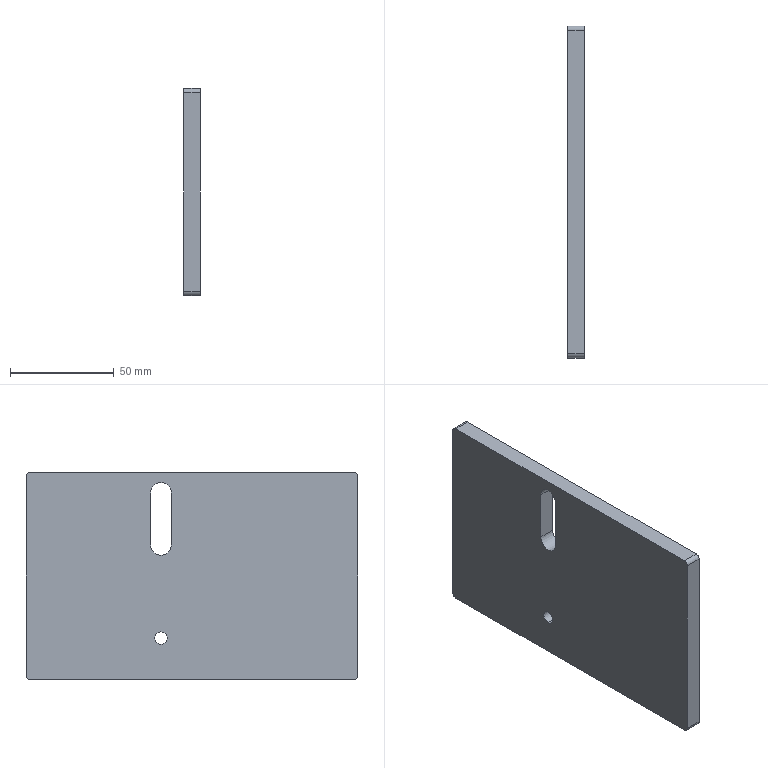Component | SolidWorks | CHEN123-AA-11-1 | 1 solid | 17 faces | box 8 x 160 x 100 mm | volume 125118 mm3 | cylinder 9 | plane 8 | commonest cylinder face diameters 4 x4 10 x3 6 x2
build123d program:
from build123d import *

# Parameters (mm, degrees)
SKETCH1_W           = 100
SKETCH1_H           = 160
BOSS_EXTRUDE1_DEPTH = 8
FILLET1_R           = 2
CUT_EXTRUDE1_DEPTH  = 95.678
SKETCH3_R           = 3
CUT_EXTRUDE2_DEPTH  = 95.678


with BuildPart() as part:
    # Sketch1 → Boss-Extrude1 (new body)
    with BuildSketch(Plane.XY):
        Rectangle(SKETCH1_W, SKETCH1_H)
    extrude(amount=BOSS_EXTRUDE1_DEPTH)

    # Fillet1
    fillet1_edges = [part.edges().sort_by_distance(p)[0] for p in [
        (50, -80, 4),
        (-50, -80, 4),
        (-50, 80, 4),
        (50, 80, 4),
    ]]
    fillet(fillet1_edges, radius=FILLET1_R)

    # Sketch2 → Cut-Extrude1 (cut, through all)
    with BuildSketch(Plane.XY.offset(8)):
        with BuildLine():
            Line((15, 10), (40, 10))
            ThreePointArc((40, 10), (45, 15), (40, 20))
            Line((40, 20), (15, 20))
            ThreePointArc((15, 20), (10, 15), (15, 10))
        make_face()
    extrude(amount=-CUT_EXTRUDE1_DEPTH, mode=Mode.SUBTRACT)

    # Sketch3 → Cut-Extrude2 (cut, through all)
    with BuildSketch(Plane(origin=(0, 0, 0), x_dir=(-1, 0, 0), z_dir=(0, 0, -1))):
        with Locations((30, 15)):
            Circle(SKETCH3_R)
    extrude(amount=-CUT_EXTRUDE2_DEPTH, mode=Mode.SUBTRACT)


solid = part.part

# Placed as in the assembly
solid = solid.moved(Location((28, -60.999, -200), (0, -90, 0)))
STEP:
#1=COLOUR_RGB('',0.7922,0.8196,0.9333);
#2=FILL_AREA_STYLE_COLOUR('',#1);
#3=FILL_AREA_STYLE('',(#2));
#4=SURFACE_STYLE_FILL_AREA(#3);
#5=SURFACE_SIDE_STYLE('',(#4));
#6=SURFACE_STYLE_USAGE(.BOTH.,#5);
#7=PRESENTATION_STYLE_ASSIGNMENT((#6));
#8=CARTESIAN_POINT('',(0.7874,-1.811,-8.937));
#9=VERTEX_POINT('',#8);
#10=CARTESIAN_POINT('',(0.7874,-1.811,-9.173));
#11=VERTEX_POINT('',#10);
#12=CARTESIAN_POINT('',(0.7874,-1.811,-9.055));
#13=DIRECTION('',(1.,0.,0.));
#14=DIRECTION('',(0.,0.,-1.));
#15=AXIS2_PLACEMENT_3D('',#12,#13,#14);
#16=CIRCLE('',#15,0.1181);
#17=EDGE_CURVE('',#9,#11,#16,.T.);
#18=ORIENTED_EDGE('',*,*,#17,.F.);
#19=CARTESIAN_POINT('',(1.102,-1.811,-8.937));
#20=VERTEX_POINT('',#19);
#21=CARTESIAN_POINT('',(0.7874,-1.811,-8.937));
#22=DIRECTION('',(1.,0.,0.));
#23=VECTOR('',#22,39.37);
#24=LINE('',#21,#23);
#25=EDGE_CURVE('',#9,#20,#24,.T.);
#26=ORIENTED_EDGE('',*,*,#25,.T.);
#27=CARTESIAN_POINT('',(1.102,-1.811,-9.173));
#28=VERTEX_POINT('',#27);
#29=CARTESIAN_POINT('',(1.102,-1.811,-9.055));
#30=DIRECTION('',(1.,0.,0.));
#31=DIRECTION('',(0.,0.,-1.));
#32=AXIS2_PLACEMENT_3D('',#29,#30,#31);
#33=CIRCLE('',#32,0.1181);
#34=EDGE_CURVE('',#20,#28,#33,.T.);
#35=ORIENTED_EDGE('',*,*,#34,.T.);
#36=CARTESIAN_POINT('',(0.7874,-1.811,-9.173));
#37=DIRECTION('',(1.,0.,0.));
#38=VECTOR('',#37,39.37);
#39=LINE('',#36,#38);
#40=EDGE_CURVE('',#11,#28,#39,.T.);
#41=ORIENTED_EDGE('',*,*,#40,.F.);
#42=EDGE_LOOP('',(#18,#26,#35,#41));
#43=FACE_OUTER_BOUND('',#42,.T.);
#44=CARTESIAN_POINT('',(0.7874,-1.811,-9.055));
#45=DIRECTION('',(1.,0.,0.));
#46=DIRECTION('',(0.,0.,-1.));
#47=AXIS2_PLACEMENT_3D('',#44,#45,#46);
#48=CYLINDRICAL_SURFACE('',#47,0.1181);
#49=ADVANCED_FACE('',(#43),#48,.F.);
#50=CARTESIAN_POINT('',(1.102,-1.811,-6.102));
#51=VERTEX_POINT('',#50);
#52=CARTESIAN_POINT('',(1.102,-1.614,-6.299));
#53=VERTEX_POINT('',#52);
#54=CARTESIAN_POINT('',(1.102,-1.811,-6.299));
#55=DIRECTION('',(-1.,0.,0.));
#56=DIRECTION('',(0.,0.,1.));
#57=AXIS2_PLACEMENT_3D('',#54,#55,#56);
#58=CIRCLE('',#57,0.1969);
#59=EDGE_CURVE('',#51,#53,#58,.T.);
#60=ORIENTED_EDGE('',*,*,#59,.F.);
#61=CARTESIAN_POINT('',(0.7874,-1.811,-6.102));
#62=VERTEX_POINT('',#61);
#63=CARTESIAN_POINT('',(1.102,-1.811,-6.102));
#64=DIRECTION('',(-1.,0.,0.));
#65=VECTOR('',#64,39.37);
#66=LINE('',#63,#65);
#67=EDGE_CURVE('',#51,#62,#66,.T.);
#68=ORIENTED_EDGE('',*,*,#67,.T.);
#69=CARTESIAN_POINT('',(0.7874,-1.614,-6.299));
#70=VERTEX_POINT('',#69);
#71=CARTESIAN_POINT('',(0.7874,-1.811,-6.299));
#72=DIRECTION('',(-1.,0.,0.));
#73=DIRECTION('',(0.,0.,1.));
#74=AXIS2_PLACEMENT_3D('',#71,#72,#73);
#75=CIRCLE('',#74,0.1969);
#76=EDGE_CURVE('',#62,#70,#75,.T.);
#77=ORIENTED_EDGE('',*,*,#76,.T.);
#78=CARTESIAN_POINT('',(1.102,-1.614,-6.299));
#79=DIRECTION('',(-1.,0.,0.));
#80=VECTOR('',#79,39.37);
#81=LINE('',#78,#80);
#82=EDGE_CURVE('',#53,#70,#81,.T.);
#83=ORIENTED_EDGE('',*,*,#82,.F.);
#84=EDGE_LOOP('',(#60,#68,#77,#83));
#85=FACE_OUTER_BOUND('',#84,.T.);
#86=CARTESIAN_POINT('',(1.102,-1.811,-6.299));
#87=DIRECTION('',(-1.,0.,0.));
#88=DIRECTION('',(0.,0.,1.));
#89=AXIS2_PLACEMENT_3D('',#86,#87,#88);
#90=CYLINDRICAL_SURFACE('',#89,0.1969);
#91=ADVANCED_FACE('',(#85),#90,.F.);
#92=CARTESIAN_POINT('',(0.7874,-5.472,-5.906));
#93=VERTEX_POINT('',#92);
#94=CARTESIAN_POINT('',(0.7874,0.6693,-5.906));
#95=VERTEX_POINT('',#94);
#96=CARTESIAN_POINT('',(0.7874,-5.551,-5.906));
#97=DIRECTION('',(0.,1.,0.));
#98=VECTOR('',#97,39.37);
#99=LINE('',#96,#98);
#100=EDGE_CURVE('',#93,#95,#99,.T.);
#101=ORIENTED_EDGE('',*,*,#100,.F.);
#102=CARTESIAN_POINT('',(1.102,-5.472,-5.906));
#103=VERTEX_POINT('',#102);
#104=CARTESIAN_POINT('',(0.7874,-5.472,-5.906));
#105=DIRECTION('',(1.,0.,0.));
#106=VECTOR('',#105,39.37);
#107=LINE('',#104,#106);
#108=EDGE_CURVE('',#93,#103,#107,.T.);
#109=ORIENTED_EDGE('',*,*,#108,.T.);
#110=CARTESIAN_POINT('',(1.102,0.6693,-5.906));
#111=VERTEX_POINT('',#110);
#112=CARTESIAN_POINT('',(1.102,-5.551,-5.906));
#113=DIRECTION('',(0.,1.,0.));
#114=VECTOR('',#113,39.37);
#115=LINE('',#112,#114);
#116=EDGE_CURVE('',#103,#111,#115,.T.);
#117=ORIENTED_EDGE('',*,*,#116,.T.);
#118=CARTESIAN_POINT('',(0.7874,0.6693,-5.906));
#119=DIRECTION('',(-1.,0.,0.));
#120=VECTOR('',#119,39.37);
#121=LINE('',#118,#120);
#122=EDGE_CURVE('',#111,#95,#121,.T.);
#123=ORIENTED_EDGE('',*,*,#122,.T.);
#124=EDGE_LOOP('',(#101,#109,#117,#123));
#125=FACE_OUTER_BOUND('',#124,.T.);
#126=CARTESIAN_POINT('',(0.7874,-5.551,-5.906));
#127=DIRECTION('',(0.,0.,-1.));
#128=DIRECTION('',(-1.,0.,0.));
#129=AXIS2_PLACEMENT_3D('',#126,#127,#128);
#130=PLANE('',#129);
#131=ADVANCED_FACE('',(#125),#130,.F.);
#132=CARTESIAN_POINT('',(0.7874,0.7481,-5.984));
#133=VERTEX_POINT('',#132);
#134=CARTESIAN_POINT('',(0.7874,0.7481,-9.764));
#135=VERTEX_POINT('',#134);
#136=CARTESIAN_POINT('',(0.7874,0.7481,-9.843));
#137=DIRECTION('',(0.,0.,-1.));
#138=VECTOR('',#137,39.37);
#139=LINE('',#136,#138);
#140=EDGE_CURVE('',#133,#135,#139,.T.);
#141=ORIENTED_EDGE('',*,*,#140,.F.);
#142=CARTESIAN_POINT('',(1.102,0.7481,-5.984));
#143=VERTEX_POINT('',#142);
#144=CARTESIAN_POINT('',(0.7874,0.7481,-5.984));
#145=DIRECTION('',(1.,0.,0.));
#146=VECTOR('',#145,39.37);
#147=LINE('',#144,#146);
#148=EDGE_CURVE('',#133,#143,#147,.T.);
#149=ORIENTED_EDGE('',*,*,#148,.T.);
#150=CARTESIAN_POINT('',(1.102,0.7481,-9.764));
#151=VERTEX_POINT('',#150);
#152=CARTESIAN_POINT('',(1.102,0.7481,-9.843));
#153=DIRECTION('',(0.,0.,-1.));
#154=VECTOR('',#153,39.37);
#155=LINE('',#152,#154);
#156=EDGE_CURVE('',#143,#151,#155,.T.);
#157=ORIENTED_EDGE('',*,*,#156,.T.);
#158=CARTESIAN_POINT('',(0.7874,0.7481,-9.764));
#159=DIRECTION('',(-1.,0.,0.));
#160=VECTOR('',#159,39.37);
#161=LINE('',#158,#160);
#162=EDGE_CURVE('',#151,#135,#161,.T.);
#163=ORIENTED_EDGE('',*,*,#162,.T.);
#164=EDGE_LOOP('',(#141,#149,#157,#163));
#165=FACE_OUTER_BOUND('',#164,.T.);
#166=CARTESIAN_POINT('',(0.7874,0.7481,-9.843));
#167=DIRECTION('',(0.,-1.,0.));
#168=DIRECTION('',(1.,0.,0.));
#169=AXIS2_PLACEMENT_3D('',#166,#167,#168);
#170=PLANE('',#169);
#171=ADVANCED_FACE('',(#165),#170,.F.);
#172=CARTESIAN_POINT('',(1.102,0.6693,-9.843));
#173=VERTEX_POINT('',#172);
#174=CARTESIAN_POINT('',(1.102,-5.472,-9.843));
#175=VERTEX_POINT('',#174);
#176=CARTESIAN_POINT('',(1.102,-5.551,-9.843));
#177=DIRECTION('',(0.,-1.,0.));
#178=VECTOR('',#177,39.37);
#179=LINE('',#176,#178);
#180=EDGE_CURVE('',#173,#175,#179,.T.);
#181=ORIENTED_EDGE('',*,*,#180,.T.);
#182=CARTESIAN_POINT('',(0.7874,-5.472,-9.843));
#183=VERTEX_POINT('',#182);
#184=CARTESIAN_POINT('',(0.7874,-5.472,-9.843));
#185=DIRECTION('',(-1.,0.,0.));
#186=VECTOR('',#185,39.37);
#187=LINE('',#184,#186);
#188=EDGE_CURVE('',#175,#183,#187,.T.);
#189=ORIENTED_EDGE('',*,*,#188,.T.);
#190=CARTESIAN_POINT('',(0.7874,0.6693,-9.843));
#191=VERTEX_POINT('',#190);
#192=CARTESIAN_POINT('',(0.7874,-5.551,-9.843));
#193=DIRECTION('',(0.,-1.,0.));
#194=VECTOR('',#193,39.37);
#195=LINE('',#192,#194);
#196=EDGE_CURVE('',#191,#183,#195,.T.);
#197=ORIENTED_EDGE('',*,*,#196,.F.);
#198=CARTESIAN_POINT('',(0.7874,0.6693,-9.843));
#199=DIRECTION('',(1.,0.,0.));
#200=VECTOR('',#199,39.37);
#201=LINE('',#198,#200);
#202=EDGE_CURVE('',#191,#173,#201,.T.);
#203=ORIENTED_EDGE('',*,*,#202,.T.);
#204=EDGE_LOOP('',(#181,#189,#197,#203));
#205=FACE_OUTER_BOUND('',#204,.T.);
#206=CARTESIAN_POINT('',(0.7874,-5.551,-9.843));
#207=DIRECTION('',(0.,0.,1.));
#208=DIRECTION('',(1.,0.,0.));
#209=AXIS2_PLACEMENT_3D('',#206,#207,#208);
#210=PLANE('',#209);
#211=ADVANCED_FACE('',(#205),#210,.F.);
#212=CARTESIAN_POINT('',(1.102,-5.551,-9.764));
#213=VERTEX_POINT('',#212);
#214=CARTESIAN_POINT('',(1.102,-5.551,-5.984));
#215=VERTEX_POINT('',#214);
#216=CARTESIAN_POINT('',(1.102,-5.551,-9.843));
#217=DIRECTION('',(0.,0.,1.));
#218=VECTOR('',#217,39.37);
#219=LINE('',#216,#218);
#220=EDGE_CURVE('',#213,#215,#219,.T.);
#221=ORIENTED_EDGE('',*,*,#220,.T.);
#222=CARTESIAN_POINT('',(0.7874,-5.551,-5.984));
#223=VERTEX_POINT('',#222);
#224=CARTESIAN_POINT('',(0.7874,-5.551,-5.984));
#225=DIRECTION('',(-1.,0.,0.));
#226=VECTOR('',#225,39.37);
#227=LINE('',#224,#226);
#228=EDGE_CURVE('',#215,#223,#227,.T.);
#229=ORIENTED_EDGE('',*,*,#228,.T.);
#230=CARTESIAN_POINT('',(0.7874,-5.551,-9.764));
#231=VERTEX_POINT('',#230);
#232=CARTESIAN_POINT('',(0.7874,-5.551,-9.843));
#233=DIRECTION('',(0.,0.,1.));
#234=VECTOR('',#233,39.37);
#235=LINE('',#232,#234);
#236=EDGE_CURVE('',#231,#223,#235,.T.);
#237=ORIENTED_EDGE('',*,*,#236,.F.);
#238=CARTESIAN_POINT('',(0.7874,-5.551,-9.764));
#239=DIRECTION('',(1.,0.,0.));
#240=VECTOR('',#239,39.37);
#241=LINE('',#238,#240);
#242=EDGE_CURVE('',#231,#213,#241,.T.);
#243=ORIENTED_EDGE('',*,*,#242,.T.);
#244=EDGE_LOOP('',(#221,#229,#237,#243));
#245=FACE_OUTER_BOUND('',#244,.T.);
#246=CARTESIAN_POINT('',(0.7874,-5.551,-9.843));
#247=DIRECTION('',(0.,1.,0.));
#248=DIRECTION('',(-1.,0.,0.));
#249=AXIS2_PLACEMENT_3D('',#246,#247,#248);
#250=PLANE('',#249);
#251=ADVANCED_FACE('',(#245),#250,.F.);
#252=CARTESIAN_POINT('',(0.7874,-1.811,-9.055));
#253=DIRECTION('',(1.,0.,0.));
#254=DIRECTION('',(0.,0.,-1.));
#255=AXIS2_PLACEMENT_3D('',#252,#253,#254);
#256=CIRCLE('',#255,0.1181);
#257=EDGE_CURVE('',#11,#9,#256,.T.);
#258=ORIENTED_EDGE('',*,*,#257,.T.);
#259=ORIENTED_EDGE('',*,*,#17,.T.);
#260=EDGE_LOOP('',(#258,#259));
#261=FACE_BOUND('',#260,.T.);
#262=CARTESIAN_POINT('',(0.7874,-1.614,-7.283));
#263=VERTEX_POINT('',#262);
#264=CARTESIAN_POINT('',(0.7874,-1.614,-6.299));
#265=DIRECTION('',(0.,0.,-1.));
#266=VECTOR('',#265,39.37);
#267=LINE('',#264,#266);
#268=EDGE_CURVE('',#70,#263,#267,.T.);
#269=ORIENTED_EDGE('',*,*,#268,.F.);
#270=ORIENTED_EDGE('',*,*,#76,.F.);
#271=CARTESIAN_POINT('',(0.7874,-2.008,-6.299));
#272=VERTEX_POINT('',#271);
#273=CARTESIAN_POINT('',(0.7874,-1.811,-6.299));
#274=DIRECTION('',(-1.,0.,0.));
#275=DIRECTION('',(0.,0.,1.));
#276=AXIS2_PLACEMENT_3D('',#273,#274,#275);
#277=CIRCLE('',#276,0.1969);
#278=EDGE_CURVE('',#272,#62,#277,.T.);
#279=ORIENTED_EDGE('',*,*,#278,.F.);
#280=CARTESIAN_POINT('',(0.7874,-2.008,-7.283));
#281=VERTEX_POINT('',#280);
#282=CARTESIAN_POINT('',(0.7874,-2.008,-7.283));
#283=DIRECTION('',(0.,0.,1.));
#284=VECTOR('',#283,39.37);
#285=LINE('',#282,#284);
#286=EDGE_CURVE('',#281,#272,#285,.T.);
#287=ORIENTED_EDGE('',*,*,#286,.F.);
#288=CARTESIAN_POINT('',(0.7874,-1.811,-7.283));
#289=DIRECTION('',(-1.,0.,0.));
#290=DIRECTION('',(0.,0.,1.));
#291=AXIS2_PLACEMENT_3D('',#288,#289,#290);
#292=CIRCLE('',#291,0.1969);
#293=EDGE_CURVE('',#263,#281,#292,.T.);
#294=ORIENTED_EDGE('',*,*,#293,.F.);
#295=EDGE_LOOP('',(#269,#270,#279,#287,#294));
#296=FACE_BOUND('',#295,.T.);
#297=ORIENTED_EDGE('',*,*,#236,.T.);
#298=CARTESIAN_POINT('',(0.7874,-5.472,-5.984));
#299=DIRECTION('',(-1.,0.,0.));
#300=DIRECTION('',(0.,0.,-1.));
#301=AXIS2_PLACEMENT_3D('',#298,#299,#300);
#302=CIRCLE('',#301,0.07874);
#303=EDGE_CURVE('',#223,#93,#302,.T.);
#304=ORIENTED_EDGE('',*,*,#303,.T.);
#305=ORIENTED_EDGE('',*,*,#100,.T.);
#306=CARTESIAN_POINT('',(0.7874,0.6693,-5.984));
#307=DIRECTION('',(-1.,0.,0.));
#308=DIRECTION('',(0.,0.,-1.));
#309=AXIS2_PLACEMENT_3D('',#306,#307,#308);
#310=CIRCLE('',#309,0.07874);
#311=EDGE_CURVE('',#95,#133,#310,.T.);
#312=ORIENTED_EDGE('',*,*,#311,.T.);
#313=ORIENTED_EDGE('',*,*,#140,.T.);
#314=CARTESIAN_POINT('',(0.7874,0.6693,-9.764));
#315=DIRECTION('',(-1.,0.,0.));
#316=DIRECTION('',(0.,0.,-1.));
#317=AXIS2_PLACEMENT_3D('',#314,#315,#316);
#318=CIRCLE('',#317,0.07874);
#319=EDGE_CURVE('',#135,#191,#318,.T.);
#320=ORIENTED_EDGE('',*,*,#319,.T.);
#321=ORIENTED_EDGE('',*,*,#196,.T.);
#322=CARTESIAN_POINT('',(0.7874,-5.472,-9.764));
#323=DIRECTION('',(-1.,0.,0.));
#324=DIRECTION('',(0.,0.,-1.));
#325=AXIS2_PLACEMENT_3D('',#322,#323,#324);
#326=CIRCLE('',#325,0.07874);
#327=EDGE_CURVE('',#183,#231,#326,.T.);
#328=ORIENTED_EDGE('',*,*,#327,.T.);
#329=EDGE_LOOP('',(#297,#304,#305,#312,#313,#320,#321,#328));
#330=FACE_OUTER_BOUND('',#329,.T.);
#331=CARTESIAN_POINT('',(0.7874,-2.402,-7.874));
#332=DIRECTION('',(1.,0.,0.));
#333=DIRECTION('',(0.,0.,-1.));
#334=AXIS2_PLACEMENT_3D('',#331,#332,#333);
#335=PLANE('',#334);
#336=ADVANCED_FACE('',(#261,#296,#330),#335,.F.);
#337=CARTESIAN_POINT('',(1.102,-1.811,-9.055));
#338=DIRECTION('',(1.,0.,0.));
#339=DIRECTION('',(0.,0.,-1.));
#340=AXIS2_PLACEMENT_3D('',#337,#338,#339);
#341=CIRCLE('',#340,0.1181);
#342=EDGE_CURVE('',#28,#20,#341,.T.);
#343=ORIENTED_EDGE('',*,*,#342,.F.);
#344=ORIENTED_EDGE('',*,*,#34,.F.);
#345=EDGE_LOOP('',(#343,#344));
#346=FACE_BOUND('',#345,.T.);
#347=CARTESIAN_POINT('',(1.102,-2.008,-6.299));
#348=VERTEX_POINT('',#347);
#349=CARTESIAN_POINT('',(1.102,-1.811,-6.299));
#350=DIRECTION('',(-1.,0.,0.));
#351=DIRECTION('',(0.,0.,1.));
#352=AXIS2_PLACEMENT_3D('',#349,#350,#351);
#353=CIRCLE('',#352,0.1969);
#354=EDGE_CURVE('',#348,#51,#353,.T.);
#355=ORIENTED_EDGE('',*,*,#354,.T.);
#356=ORIENTED_EDGE('',*,*,#59,.T.);
#357=CARTESIAN_POINT('',(1.102,-1.614,-7.283));
#358=VERTEX_POINT('',#357);
#359=CARTESIAN_POINT('',(1.102,-1.614,-6.299));
#360=DIRECTION('',(0.,0.,-1.));
#361=VECTOR('',#360,39.37);
#362=LINE('',#359,#361);
#363=EDGE_CURVE('',#53,#358,#362,.T.);
#364=ORIENTED_EDGE('',*,*,#363,.T.);
#365=CARTESIAN_POINT('',(1.102,-2.008,-7.283));
#366=VERTEX_POINT('',#365);
#367=CARTESIAN_POINT('',(1.102,-1.811,-7.283));
#368=DIRECTION('',(-1.,0.,0.));
#369=DIRECTION('',(0.,0.,1.));
#370=AXIS2_PLACEMENT_3D('',#367,#368,#369);
#371=CIRCLE('',#370,0.1969);
#372=EDGE_CURVE('',#358,#366,#371,.T.);
#373=ORIENTED_EDGE('',*,*,#372,.T.);
#374=CARTESIAN_POINT('',(1.102,-2.008,-7.283));
#375=DIRECTION('',(0.,0.,1.));
#376=VECTOR('',#375,39.37);
#377=LINE('',#374,#376);
#378=EDGE_CURVE('',#366,#348,#377,.T.);
#379=ORIENTED_EDGE('',*,*,#378,.T.);
#380=EDGE_LOOP('',(#355,#356,#364,#373,#379));
#381=FACE_BOUND('',#380,.T.);
#382=ORIENTED_EDGE('',*,*,#116,.F.);
#383=CARTESIAN_POINT('',(1.102,-5.472,-5.984));
#384=DIRECTION('',(1.,0.,0.));
#385=DIRECTION('',(0.,0.,-1.));
#386=AXIS2_PLACEMENT_3D('',#383,#384,#385);
#387=CIRCLE('',#386,0.07874);
#388=EDGE_CURVE('',#103,#215,#387,.T.);
#389=ORIENTED_EDGE('',*,*,#388,.T.);
#390=ORIENTED_EDGE('',*,*,#220,.F.);
#391=CARTESIAN_POINT('',(1.102,-5.472,-9.764));
#392=DIRECTION('',(1.,0.,0.));
#393=DIRECTION('',(0.,0.,-1.));
#394=AXIS2_PLACEMENT_3D('',#391,#392,#393);
#395=CIRCLE('',#394,0.07874);
#396=EDGE_CURVE('',#213,#175,#395,.T.);
#397=ORIENTED_EDGE('',*,*,#396,.T.);
#398=ORIENTED_EDGE('',*,*,#180,.F.);
#399=CARTESIAN_POINT('',(1.102,0.6693,-9.764));
#400=DIRECTION('',(1.,0.,0.));
#401=DIRECTION('',(0.,0.,-1.));
#402=AXIS2_PLACEMENT_3D('',#399,#400,#401);
#403=CIRCLE('',#402,0.07874);
#404=EDGE_CURVE('',#173,#151,#403,.T.);
#405=ORIENTED_EDGE('',*,*,#404,.T.);
#406=ORIENTED_EDGE('',*,*,#156,.F.);
#407=CARTESIAN_POINT('',(1.102,0.6693,-5.984));
#408=DIRECTION('',(1.,0.,0.));
#409=DIRECTION('',(0.,0.,-1.));
#410=AXIS2_PLACEMENT_3D('',#407,#408,#409);
#411=CIRCLE('',#410,0.07874);
#412=EDGE_CURVE('',#143,#111,#411,.T.);
#413=ORIENTED_EDGE('',*,*,#412,.T.);
#414=EDGE_LOOP('',(#382,#389,#390,#397,#398,#405,#406,#413));
#415=FACE_OUTER_BOUND('',#414,.T.);
#416=CARTESIAN_POINT('',(1.102,-2.402,-7.874));
#417=DIRECTION('',(1.,0.,0.));
#418=DIRECTION('',(0.,0.,-1.));
#419=AXIS2_PLACEMENT_3D('',#416,#417,#418);
#420=PLANE('',#419);
#421=ADVANCED_FACE('',(#346,#381,#415),#420,.T.);
#422=ORIENTED_EDGE('',*,*,#303,.F.);
#423=ORIENTED_EDGE('',*,*,#228,.F.);
#424=ORIENTED_EDGE('',*,*,#388,.F.);
#425=ORIENTED_EDGE('',*,*,#108,.F.);
#426=EDGE_LOOP('',(#422,#423,#424,#425));
#427=FACE_OUTER_BOUND('',#426,.T.);
#428=CARTESIAN_POINT('',(0.7874,-5.472,-5.984));
#429=DIRECTION('',(1.,0.,0.));
#430=DIRECTION('',(0.,0.,-1.));
#431=AXIS2_PLACEMENT_3D('',#428,#429,#430);
#432=CYLINDRICAL_SURFACE('',#431,0.07874);
#433=ADVANCED_FACE('',(#427),#432,.T.);
#434=ORIENTED_EDGE('',*,*,#327,.F.);
#435=ORIENTED_EDGE('',*,*,#188,.F.);
#436=ORIENTED_EDGE('',*,*,#396,.F.);
#437=ORIENTED_EDGE('',*,*,#242,.F.);
#438=EDGE_LOOP('',(#434,#435,#436,#437));
#439=FACE_OUTER_BOUND('',#438,.T.);
#440=CARTESIAN_POINT('',(0.7874,-5.472,-9.764));
#441=DIRECTION('',(1.,0.,0.));
#442=DIRECTION('',(0.,0.,-1.));
#443=AXIS2_PLACEMENT_3D('',#440,#441,#442);
#444=CYLINDRICAL_SURFACE('',#443,0.07874);
#445=ADVANCED_FACE('',(#439),#444,.T.);
#446=ORIENTED_EDGE('',*,*,#311,.F.);
#447=ORIENTED_EDGE('',*,*,#122,.F.);
#448=ORIENTED_EDGE('',*,*,#412,.F.);
#449=ORIENTED_EDGE('',*,*,#148,.F.);
#450=EDGE_LOOP('',(#446,#447,#448,#449));
#451=FACE_OUTER_BOUND('',#450,.T.);
#452=CARTESIAN_POINT('',(0.7874,0.6693,-5.984));
#453=DIRECTION('',(1.,0.,0.));
#454=DIRECTION('',(0.,0.,-1.));
#455=AXIS2_PLACEMENT_3D('',#452,#453,#454);
#456=CYLINDRICAL_SURFACE('',#455,0.07874);
#457=ADVANCED_FACE('',(#451),#456,.T.);
#458=ORIENTED_EDGE('',*,*,#319,.F.);
#459=ORIENTED_EDGE('',*,*,#162,.F.);
#460=ORIENTED_EDGE('',*,*,#404,.F.);
#461=ORIENTED_EDGE('',*,*,#202,.F.);
#462=EDGE_LOOP('',(#458,#459,#460,#461));
#463=FACE_OUTER_BOUND('',#462,.T.);
#464=CARTESIAN_POINT('',(0.7874,0.6693,-9.764));
#465=DIRECTION('',(1.,0.,0.));
#466=DIRECTION('',(0.,0.,-1.));
#467=AXIS2_PLACEMENT_3D('',#464,#465,#466);
#468=CYLINDRICAL_SURFACE('',#467,0.07874);
#469=ADVANCED_FACE('',(#463),#468,.T.);
#470=ORIENTED_EDGE('',*,*,#67,.F.);
#471=ORIENTED_EDGE('',*,*,#354,.F.);
#472=CARTESIAN_POINT('',(1.102,-2.008,-6.299));
#473=DIRECTION('',(-1.,0.,0.));
#474=VECTOR('',#473,39.37);
#475=LINE('',#472,#474);
#476=EDGE_CURVE('',#348,#272,#475,.T.);
#477=ORIENTED_EDGE('',*,*,#476,.T.);
#478=ORIENTED_EDGE('',*,*,#278,.T.);
#479=EDGE_LOOP('',(#470,#471,#477,#478));
#480=FACE_OUTER_BOUND('',#479,.T.);
#481=CARTESIAN_POINT('',(1.102,-1.811,-6.299));
#482=DIRECTION('',(-1.,0.,0.));
#483=DIRECTION('',(0.,0.,1.));
#484=AXIS2_PLACEMENT_3D('',#481,#482,#483);
#485=CYLINDRICAL_SURFACE('',#484,0.1969);
#486=ADVANCED_FACE('',(#480),#485,.F.);
#487=ORIENTED_EDGE('',*,*,#286,.T.);
#488=ORIENTED_EDGE('',*,*,#476,.F.);
#489=ORIENTED_EDGE('',*,*,#378,.F.);
#490=CARTESIAN_POINT('',(1.102,-2.008,-7.283));
#491=DIRECTION('',(-1.,0.,0.));
#492=VECTOR('',#491,39.37);
#493=LINE('',#490,#492);
#494=EDGE_CURVE('',#366,#281,#493,.T.);
#495=ORIENTED_EDGE('',*,*,#494,.T.);
#496=EDGE_LOOP('',(#487,#488,#489,#495));
#497=FACE_OUTER_BOUND('',#496,.T.);
#498=CARTESIAN_POINT('',(1.102,-2.008,-7.283));
#499=DIRECTION('',(0.,-1.,0.));
#500=DIRECTION('',(0.,0.,1.));
#501=AXIS2_PLACEMENT_3D('',#498,#499,#500);
#502=PLANE('',#501);
#503=ADVANCED_FACE('',(#497),#502,.F.);
#504=ORIENTED_EDGE('',*,*,#293,.T.);
#505=ORIENTED_EDGE('',*,*,#494,.F.);
#506=ORIENTED_EDGE('',*,*,#372,.F.);
#507=CARTESIAN_POINT('',(1.102,-1.614,-7.283));
#508=DIRECTION('',(-1.,0.,0.));
#509=VECTOR('',#508,39.37);
#510=LINE('',#507,#509);
#511=EDGE_CURVE('',#358,#263,#510,.T.);
#512=ORIENTED_EDGE('',*,*,#511,.T.);
#513=EDGE_LOOP('',(#504,#505,#506,#512));
#514=FACE_OUTER_BOUND('',#513,.T.);
#515=CARTESIAN_POINT('',(1.102,-1.811,-7.283));
#516=DIRECTION('',(-1.,0.,0.));
#517=DIRECTION('',(0.,0.,1.));
#518=AXIS2_PLACEMENT_3D('',#515,#516,#517);
#519=CYLINDRICAL_SURFACE('',#518,0.1969);
#520=ADVANCED_FACE('',(#514),#519,.F.);
#521=ORIENTED_EDGE('',*,*,#268,.T.);
#522=ORIENTED_EDGE('',*,*,#511,.F.);
#523=ORIENTED_EDGE('',*,*,#363,.F.);
#524=ORIENTED_EDGE('',*,*,#82,.T.);
#525=EDGE_LOOP('',(#521,#522,#523,#524));
#526=FACE_OUTER_BOUND('',#525,.T.);
#527=CARTESIAN_POINT('',(1.102,-1.614,-6.299));
#528=DIRECTION('',(0.,1.,0.));
#529=DIRECTION('',(-1.,0.,0.));
#530=AXIS2_PLACEMENT_3D('',#527,#528,#529);
#531=PLANE('',#530);
#532=ADVANCED_FACE('',(#526),#531,.F.);
#533=ORIENTED_EDGE('',*,*,#25,.F.);
#534=ORIENTED_EDGE('',*,*,#257,.F.);
#535=ORIENTED_EDGE('',*,*,#40,.T.);
#536=ORIENTED_EDGE('',*,*,#342,.T.);
#537=EDGE_LOOP('',(#533,#534,#535,#536));
#538=FACE_OUTER_BOUND('',#537,.T.);
#539=CARTESIAN_POINT('',(0.7874,-1.811,-9.055));
#540=DIRECTION('',(1.,0.,0.));
#541=DIRECTION('',(0.,0.,-1.));
#542=AXIS2_PLACEMENT_3D('',#539,#540,#541);
#543=CYLINDRICAL_SURFACE('',#542,0.1181);
#544=ADVANCED_FACE('',(#538),#543,.F.);
#545=CLOSED_SHELL('',(#49,#91,#131,#171,#211,#251,#336,#421,#433,#445,#457,#469,#486,#503,#520,#532,#544));
#546=MANIFOLD_SOLID_BREP('',#545);
#547=STYLED_ITEM('',(#7),#546);
#548=(LENGTH_UNIT()NAMED_UNIT(*)SI_UNIT($,.METRE.));
#549=LENGTH_MEASURE_WITH_UNIT(LENGTH_MEASURE(0.0254),#548);
#550=DIMENSIONAL_EXPONENTS(1.,0.,0.,0.,0.,0.,0.);
#551=(CONVERSION_BASED_UNIT('',#549)LENGTH_UNIT()NAMED_UNIT(#550));
#552=UNCERTAINTY_MEASURE_WITH_UNIT(LENGTH_MEASURE(0.00001),#551,'','');
#553=(NAMED_UNIT(*)PLANE_ANGLE_UNIT()SI_UNIT($,.RADIAN.));
#554=(NAMED_UNIT(*)SI_UNIT($,.STERADIAN.)SOLID_ANGLE_UNIT());
#555=(GEOMETRIC_REPRESENTATION_CONTEXT(3)GLOBAL_UNCERTAINTY_ASSIGNED_CONTEXT((#552))GLOBAL_UNIT_ASSIGNED_CONTEXT((#551,#553,#554))REPRESENTATION_CONTEXT('',''));
#556=MECHANICAL_DESIGN_GEOMETRIC_PRESENTATION_REPRESENTATION('',(#547),#555);
#557=CARTESIAN_POINT('',(0.,0.,0.));
#558=DIRECTION('',(0.,0.,1.));
#559=DIRECTION('',(1.,0.,0.));
#560=AXIS2_PLACEMENT_3D('',#557,#558,#559);
#561=(LENGTH_UNIT()NAMED_UNIT(*)SI_UNIT($,.METRE.));
#562=LENGTH_MEASURE_WITH_UNIT(LENGTH_MEASURE(0.0254),#561);
#563=DIMENSIONAL_EXPONENTS(1.,0.,0.,0.,0.,0.,0.);
#564=(CONVERSION_BASED_UNIT('',#562)LENGTH_UNIT()NAMED_UNIT(#563));
#565=UNCERTAINTY_MEASURE_WITH_UNIT(LENGTH_MEASURE(0.00001),#564,'','');
#566=(NAMED_UNIT(*)PLANE_ANGLE_UNIT()SI_UNIT($,.RADIAN.));
#567=(NAMED_UNIT(*)SI_UNIT($,.STERADIAN.)SOLID_ANGLE_UNIT());
#568=(GEOMETRIC_REPRESENTATION_CONTEXT(3)GLOBAL_UNCERTAINTY_ASSIGNED_CONTEXT((#565))GLOBAL_UNIT_ASSIGNED_CONTEXT((#564,#566,#567))REPRESENTATION_CONTEXT('',''));
#569=ADVANCED_BREP_SHAPE_REPRESENTATION('',(#546,#560),#568);
#570=PRESENTATION_LAYER_ASSIGNMENT('','',(#547));